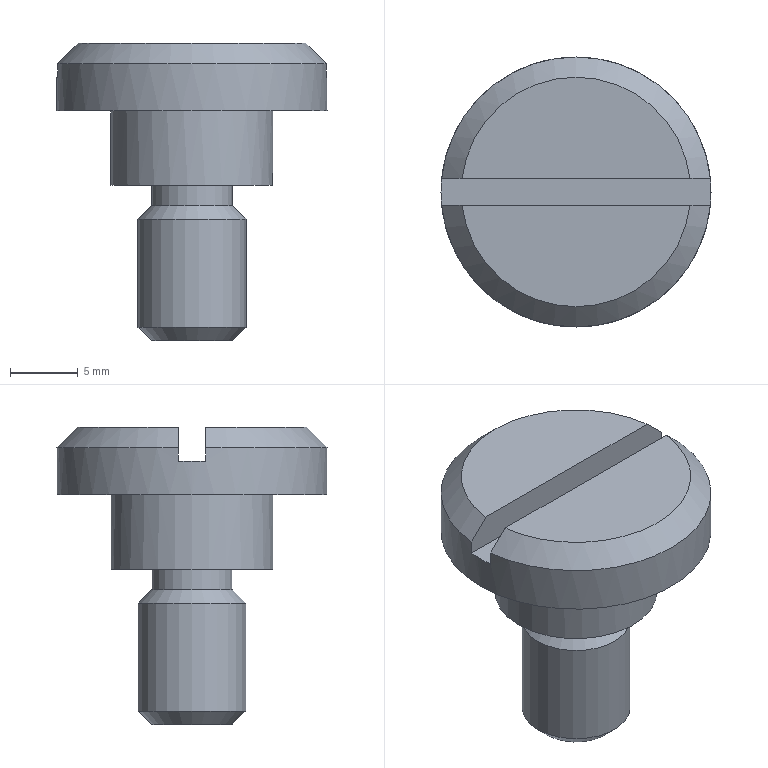Component | NX | DRILL_BUSH_SCREW_3 | 1 solid | 16 faces | volume 2552 mm3 | plane 8 | cylinder 4 | cone 4 | commonest cylinder face diameters 8 x1 6 x1 12 x1 20 x1